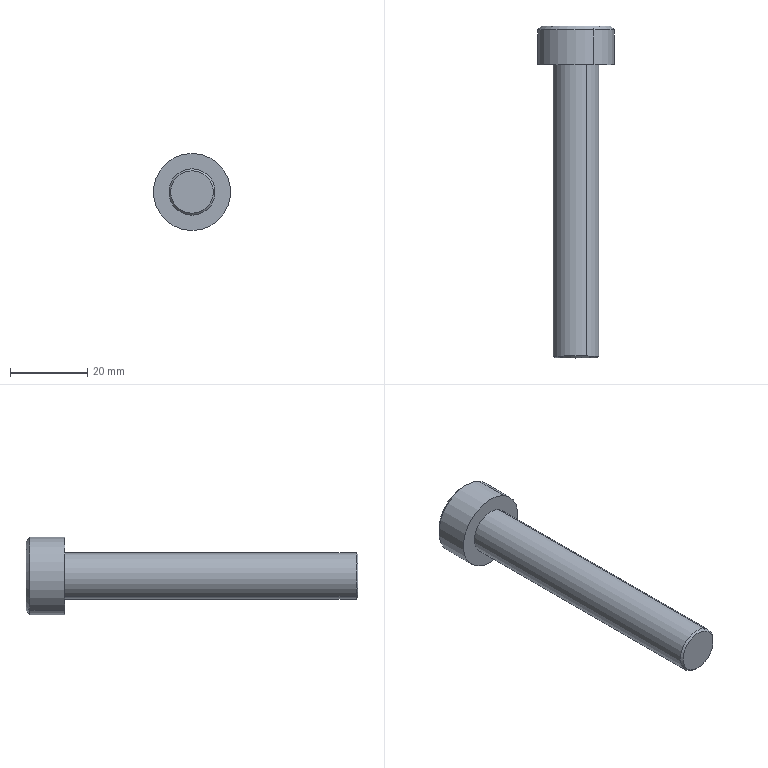Component | SolidWorks | DirectPressureVerticalSeal-1_PinShaft-1 | 1 solid | 11 faces | box 20 x 86 x 20 mm | volume 11702 mm3 | cylinder 4 | cone 4 | plane 3 | commonest cylinder face diameters 12 x2 20 x2
STEP:
#1=COLOUR_RGB('',0.7922,0.8196,0.9333);
#2=FILL_AREA_STYLE_COLOUR('',#1);
#3=FILL_AREA_STYLE('',(#2));
#4=SURFACE_STYLE_FILL_AREA(#3);
#5=SURFACE_SIDE_STYLE('',(#4));
#6=SURFACE_STYLE_USAGE(.BOTH.,#5);
#7=PRESENTATION_STYLE_ASSIGNMENT((#6));
#8=CARTESIAN_POINT('',(-4.959,8.243,11.567));
#9=VERTEX_POINT('',#8);
#10=CARTESIAN_POINT('',(-5.179,8.243,11.149));
#11=VERTEX_POINT('',#10);
#12=CARTESIAN_POINT('',(-5.069,8.243,11.358));
#13=DIRECTION('',(0.,1.,0.));
#14=DIRECTION('',(0.4655,0.,0.885));
#15=AXIS2_PLACEMENT_3D('',#12,#13,#14);
#16=CIRCLE('',#15,0.2362);
#17=EDGE_CURVE('',#9,#11,#16,.T.);
#18=ORIENTED_EDGE('',*,*,#17,.T.);
#19=CARTESIAN_POINT('',(-5.179,11.215,11.149));
#20=VERTEX_POINT('',#19);
#21=CARTESIAN_POINT('',(-5.179,11.609,11.149));
#22=DIRECTION('',(0.,1.,0.));
#23=VECTOR('',#22,39.37);
#24=LINE('',#21,#23);
#25=EDGE_CURVE('',#11,#20,#24,.T.);
#26=ORIENTED_EDGE('',*,*,#25,.T.);
#27=CARTESIAN_POINT('',(-4.959,11.215,11.567));
#28=VERTEX_POINT('',#27);
#29=CARTESIAN_POINT('',(-5.069,11.215,11.358));
#30=DIRECTION('',(-0.,-1.,-0.));
#31=DIRECTION('',(0.4655,0.,0.885));
#32=AXIS2_PLACEMENT_3D('',#29,#30,#31);
#33=CIRCLE('',#32,0.2362);
#34=EDGE_CURVE('',#20,#28,#33,.T.);
#35=ORIENTED_EDGE('',*,*,#34,.T.);
#36=CARTESIAN_POINT('',(-4.959,11.609,11.567));
#37=DIRECTION('',(0.,1.,0.));
#38=VECTOR('',#37,39.37);
#39=LINE('',#36,#38);
#40=EDGE_CURVE('',#9,#28,#39,.T.);
#41=ORIENTED_EDGE('',*,*,#40,.F.);
#42=EDGE_LOOP('',(#18,#26,#35,#41));
#43=FACE_OUTER_BOUND('',#42,.T.);
#44=CARTESIAN_POINT('',(-5.069,11.609,11.358));
#45=DIRECTION('',(0.,1.,0.));
#46=DIRECTION('',(0.4655,0.,0.885));
#47=AXIS2_PLACEMENT_3D('',#44,#45,#46);
#48=CYLINDRICAL_SURFACE('',#47,0.2362);
#49=ADVANCED_FACE('',(#43),#48,.T.);
#50=CARTESIAN_POINT('',(-4.968,8.223,11.55));
#51=VERTEX_POINT('',#50);
#52=CARTESIAN_POINT('',(-5.17,8.223,11.167));
#53=VERTEX_POINT('',#52);
#54=CARTESIAN_POINT('',(-5.069,8.223,11.358));
#55=DIRECTION('',(0.,1.,0.));
#56=DIRECTION('',(0.4655,0.,0.885));
#57=AXIS2_PLACEMENT_3D('',#54,#55,#56);
#58=CIRCLE('',#57,0.2165);
#59=EDGE_CURVE('',#51,#53,#58,.T.);
#60=ORIENTED_EDGE('',*,*,#59,.T.);
#61=CARTESIAN_POINT('',(-5.179,8.243,11.149));
#62=DIRECTION('',(-0.3292,0.7071,-0.6258));
#63=VECTOR('',#62,39.37);
#64=LINE('',#61,#63);
#65=EDGE_CURVE('',#53,#11,#64,.T.);
#66=ORIENTED_EDGE('',*,*,#65,.T.);
#67=ORIENTED_EDGE('',*,*,#17,.F.);
#68=CARTESIAN_POINT('',(-4.959,8.243,11.567));
#69=DIRECTION('',(0.3292,0.7071,0.6258));
#70=VECTOR('',#69,39.37);
#71=LINE('',#68,#70);
#72=EDGE_CURVE('',#51,#9,#71,.T.);
#73=ORIENTED_EDGE('',*,*,#72,.F.);
#74=EDGE_LOOP('',(#60,#66,#67,#73));
#75=FACE_OUTER_BOUND('',#74,.T.);
#76=CARTESIAN_POINT('',(-5.069,8.243,11.358));
#77=DIRECTION('',(0.,1.,0.));
#78=DIRECTION('',(0.4655,0.,0.885));
#79=AXIS2_PLACEMENT_3D('',#76,#77,#78);
#80=CONICAL_SURFACE('',#79,0.2362,0.7854);
#81=ADVANCED_FACE('',(#75),#80,.T.);
#82=CARTESIAN_POINT('',(-4.885,11.215,11.707));
#83=VERTEX_POINT('',#82);
#84=CARTESIAN_POINT('',(-5.252,11.215,11.01));
#85=VERTEX_POINT('',#84);
#86=CARTESIAN_POINT('',(-5.069,11.215,11.358));
#87=DIRECTION('',(0.,1.,0.));
#88=DIRECTION('',(0.4655,0.,0.885));
#89=AXIS2_PLACEMENT_3D('',#86,#87,#88);
#90=CIRCLE('',#89,0.3937);
#91=EDGE_CURVE('',#83,#85,#90,.T.);
#92=ORIENTED_EDGE('',*,*,#91,.T.);
#93=CARTESIAN_POINT('',(-5.252,11.57,11.01));
#94=VERTEX_POINT('',#93);
#95=CARTESIAN_POINT('',(-5.252,11.609,11.01));
#96=DIRECTION('',(0.,1.,0.));
#97=VECTOR('',#96,39.37);
#98=LINE('',#95,#97);
#99=EDGE_CURVE('',#85,#94,#98,.T.);
#100=ORIENTED_EDGE('',*,*,#99,.T.);
#101=CARTESIAN_POINT('',(-4.885,11.57,11.707));
#102=VERTEX_POINT('',#101);
#103=CARTESIAN_POINT('',(-5.069,11.57,11.358));
#104=DIRECTION('',(-0.,-1.,-0.));
#105=DIRECTION('',(0.4655,0.,0.885));
#106=AXIS2_PLACEMENT_3D('',#103,#104,#105);
#107=CIRCLE('',#106,0.3937);
#108=EDGE_CURVE('',#94,#102,#107,.T.);
#109=ORIENTED_EDGE('',*,*,#108,.T.);
#110=CARTESIAN_POINT('',(-4.885,11.609,11.707));
#111=DIRECTION('',(0.,1.,0.));
#112=VECTOR('',#111,39.37);
#113=LINE('',#110,#112);
#114=EDGE_CURVE('',#83,#102,#113,.T.);
#115=ORIENTED_EDGE('',*,*,#114,.F.);
#116=EDGE_LOOP('',(#92,#100,#109,#115));
#117=FACE_OUTER_BOUND('',#116,.T.);
#118=CARTESIAN_POINT('',(-5.069,11.609,11.358));
#119=DIRECTION('',(0.,1.,0.));
#120=DIRECTION('',(0.4655,0.,0.885));
#121=AXIS2_PLACEMENT_3D('',#118,#119,#120);
#122=CYLINDRICAL_SURFACE('',#121,0.3937);
#123=ADVANCED_FACE('',(#117),#122,.T.);
#124=CARTESIAN_POINT('',(-5.234,11.609,11.045));
#125=VERTEX_POINT('',#124);
#126=CARTESIAN_POINT('',(-4.904,11.609,11.672));
#127=VERTEX_POINT('',#126);
#128=CARTESIAN_POINT('',(-5.069,11.609,11.358));
#129=DIRECTION('',(-0.,-1.,-0.));
#130=DIRECTION('',(-0.4655,0.,-0.885));
#131=AXIS2_PLACEMENT_3D('',#128,#129,#130);
#132=CIRCLE('',#131,0.3543);
#133=EDGE_CURVE('',#125,#127,#132,.T.);
#134=ORIENTED_EDGE('',*,*,#133,.T.);
#135=CARTESIAN_POINT('',(-4.885,11.57,11.707));
#136=DIRECTION('',(0.3292,-0.7071,0.6258));
#137=VECTOR('',#136,39.37);
#138=LINE('',#135,#137);
#139=EDGE_CURVE('',#127,#102,#138,.T.);
#140=ORIENTED_EDGE('',*,*,#139,.T.);
#141=ORIENTED_EDGE('',*,*,#108,.F.);
#142=CARTESIAN_POINT('',(-5.252,11.57,11.01));
#143=DIRECTION('',(-0.3292,-0.7071,-0.6258));
#144=VECTOR('',#143,39.37);
#145=LINE('',#142,#144);
#146=EDGE_CURVE('',#125,#94,#145,.T.);
#147=ORIENTED_EDGE('',*,*,#146,.F.);
#148=EDGE_LOOP('',(#134,#140,#141,#147));
#149=FACE_OUTER_BOUND('',#148,.T.);
#150=CARTESIAN_POINT('',(-5.069,11.57,11.358));
#151=DIRECTION('',(-0.,-1.,-0.));
#152=DIRECTION('',(-0.4655,0.,-0.885));
#153=AXIS2_PLACEMENT_3D('',#150,#151,#152);
#154=CONICAL_SURFACE('',#153,0.3937,0.7854);
#155=ADVANCED_FACE('',(#149),#154,.T.);
#156=ORIENTED_EDGE('',*,*,#25,.F.);
#157=CARTESIAN_POINT('',(-5.069,8.243,11.358));
#158=DIRECTION('',(0.,1.,0.));
#159=DIRECTION('',(0.4655,0.,0.885));
#160=AXIS2_PLACEMENT_3D('',#157,#158,#159);
#161=CIRCLE('',#160,0.2362);
#162=EDGE_CURVE('',#11,#9,#161,.T.);
#163=ORIENTED_EDGE('',*,*,#162,.T.);
#164=ORIENTED_EDGE('',*,*,#40,.T.);
#165=CARTESIAN_POINT('',(-5.069,11.215,11.358));
#166=DIRECTION('',(-0.,-1.,-0.));
#167=DIRECTION('',(0.4655,0.,0.885));
#168=AXIS2_PLACEMENT_3D('',#165,#166,#167);
#169=CIRCLE('',#168,0.2362);
#170=EDGE_CURVE('',#28,#20,#169,.T.);
#171=ORIENTED_EDGE('',*,*,#170,.T.);
#172=EDGE_LOOP('',(#156,#163,#164,#171));
#173=FACE_OUTER_BOUND('',#172,.T.);
#174=CARTESIAN_POINT('',(-5.069,11.609,11.358));
#175=DIRECTION('',(0.,1.,0.));
#176=DIRECTION('',(0.4655,0.,0.885));
#177=AXIS2_PLACEMENT_3D('',#174,#175,#176);
#178=CYLINDRICAL_SURFACE('',#177,0.2362);
#179=ADVANCED_FACE('',(#173),#178,.T.);
#180=ORIENTED_EDGE('',*,*,#91,.F.);
#181=CARTESIAN_POINT('',(-5.069,11.215,11.358));
#182=DIRECTION('',(0.,1.,0.));
#183=DIRECTION('',(0.4655,0.,0.885));
#184=AXIS2_PLACEMENT_3D('',#181,#182,#183);
#185=CIRCLE('',#184,0.3937);
#186=EDGE_CURVE('',#85,#83,#185,.T.);
#187=ORIENTED_EDGE('',*,*,#186,.F.);
#188=EDGE_LOOP('',(#180,#187));
#189=FACE_OUTER_BOUND('',#188,.T.);
#190=ORIENTED_EDGE('',*,*,#170,.F.);
#191=ORIENTED_EDGE('',*,*,#34,.F.);
#192=EDGE_LOOP('',(#190,#191));
#193=FACE_BOUND('',#192,.T.);
#194=CARTESIAN_POINT('',(-4.86,11.215,11.248));
#195=DIRECTION('',(0.,1.,0.));
#196=DIRECTION('',(0.4655,-0.,0.885));
#197=AXIS2_PLACEMENT_3D('',#194,#195,#196);
#198=PLANE('',#197);
#199=ADVANCED_FACE('',(#189,#193),#198,.F.);
#200=ORIENTED_EDGE('',*,*,#65,.F.);
#201=CARTESIAN_POINT('',(-5.069,8.223,11.358));
#202=DIRECTION('',(0.,1.,0.));
#203=DIRECTION('',(0.4655,0.,0.885));
#204=AXIS2_PLACEMENT_3D('',#201,#202,#203);
#205=CIRCLE('',#204,0.2165);
#206=EDGE_CURVE('',#53,#51,#205,.T.);
#207=ORIENTED_EDGE('',*,*,#206,.T.);
#208=ORIENTED_EDGE('',*,*,#72,.T.);
#209=ORIENTED_EDGE('',*,*,#162,.F.);
#210=EDGE_LOOP('',(#200,#207,#208,#209));
#211=FACE_OUTER_BOUND('',#210,.T.);
#212=CARTESIAN_POINT('',(-5.069,8.243,11.358));
#213=DIRECTION('',(0.,1.,0.));
#214=DIRECTION('',(0.4655,0.,0.885));
#215=AXIS2_PLACEMENT_3D('',#212,#213,#214);
#216=CONICAL_SURFACE('',#215,0.2362,0.7854);
#217=ADVANCED_FACE('',(#211),#216,.T.);
#218=ORIENTED_EDGE('',*,*,#99,.F.);
#219=ORIENTED_EDGE('',*,*,#186,.T.);
#220=ORIENTED_EDGE('',*,*,#114,.T.);
#221=CARTESIAN_POINT('',(-5.069,11.57,11.358));
#222=DIRECTION('',(-0.,-1.,-0.));
#223=DIRECTION('',(0.4655,0.,0.885));
#224=AXIS2_PLACEMENT_3D('',#221,#222,#223);
#225=CIRCLE('',#224,0.3937);
#226=EDGE_CURVE('',#102,#94,#225,.T.);
#227=ORIENTED_EDGE('',*,*,#226,.T.);
#228=EDGE_LOOP('',(#218,#219,#220,#227));
#229=FACE_OUTER_BOUND('',#228,.T.);
#230=CARTESIAN_POINT('',(-5.069,11.609,11.358));
#231=DIRECTION('',(0.,1.,0.));
#232=DIRECTION('',(0.4655,0.,0.885));
#233=AXIS2_PLACEMENT_3D('',#230,#231,#232);
#234=CYLINDRICAL_SURFACE('',#233,0.3937);
#235=ADVANCED_FACE('',(#229),#234,.T.);
#236=ORIENTED_EDGE('',*,*,#59,.F.);
#237=ORIENTED_EDGE('',*,*,#206,.F.);
#238=EDGE_LOOP('',(#236,#237));
#239=FACE_OUTER_BOUND('',#238,.T.);
#240=CARTESIAN_POINT('',(-5.069,8.223,11.358));
#241=DIRECTION('',(0.,1.,0.));
#242=DIRECTION('',(0.4655,-0.,0.885));
#243=AXIS2_PLACEMENT_3D('',#240,#241,#242);
#244=PLANE('',#243);
#245=ADVANCED_FACE('',(#239),#244,.F.);
#246=ORIENTED_EDGE('',*,*,#139,.F.);
#247=CARTESIAN_POINT('',(-5.069,11.609,11.358));
#248=DIRECTION('',(-0.,-1.,-0.));
#249=DIRECTION('',(-0.4655,0.,-0.885));
#250=AXIS2_PLACEMENT_3D('',#247,#248,#249);
#251=CIRCLE('',#250,0.3543);
#252=EDGE_CURVE('',#127,#125,#251,.T.);
#253=ORIENTED_EDGE('',*,*,#252,.T.);
#254=ORIENTED_EDGE('',*,*,#146,.T.);
#255=ORIENTED_EDGE('',*,*,#226,.F.);
#256=EDGE_LOOP('',(#246,#253,#254,#255));
#257=FACE_OUTER_BOUND('',#256,.T.);
#258=CARTESIAN_POINT('',(-5.069,11.57,11.358));
#259=DIRECTION('',(-0.,-1.,-0.));
#260=DIRECTION('',(-0.4655,0.,-0.885));
#261=AXIS2_PLACEMENT_3D('',#258,#259,#260);
#262=CONICAL_SURFACE('',#261,0.3937,0.7854);
#263=ADVANCED_FACE('',(#257),#262,.T.);
#264=ORIENTED_EDGE('',*,*,#133,.F.);
#265=ORIENTED_EDGE('',*,*,#252,.F.);
#266=EDGE_LOOP('',(#264,#265));
#267=FACE_OUTER_BOUND('',#266,.T.);
#268=CARTESIAN_POINT('',(-4.755,11.609,11.193));
#269=DIRECTION('',(-0.,-1.,-0.));
#270=DIRECTION('',(-0.4655,0.,-0.885));
#271=AXIS2_PLACEMENT_3D('',#268,#269,#270);
#272=PLANE('',#271);
#273=ADVANCED_FACE('',(#267),#272,.F.);
#274=CLOSED_SHELL('',(#49,#81,#123,#155,#179,#199,#217,#235,#245,#263,#273));
#275=MANIFOLD_SOLID_BREP('',#274);
#276=STYLED_ITEM('',(#7),#275);
#277=(LENGTH_UNIT()NAMED_UNIT(*)SI_UNIT($,.METRE.));
#278=LENGTH_MEASURE_WITH_UNIT(LENGTH_MEASURE(0.0254),#277);
#279=DIMENSIONAL_EXPONENTS(1.,0.,0.,0.,0.,0.,0.);
#280=(CONVERSION_BASED_UNIT('',#278)LENGTH_UNIT()NAMED_UNIT(#279));
#281=UNCERTAINTY_MEASURE_WITH_UNIT(LENGTH_MEASURE(0.00001),#280,'','');
#282=(NAMED_UNIT(*)PLANE_ANGLE_UNIT()SI_UNIT($,.RADIAN.));
#283=(NAMED_UNIT(*)SI_UNIT($,.STERADIAN.)SOLID_ANGLE_UNIT());
#284=(GEOMETRIC_REPRESENTATION_CONTEXT(3)GLOBAL_UNCERTAINTY_ASSIGNED_CONTEXT((#281))GLOBAL_UNIT_ASSIGNED_CONTEXT((#280,#282,#283))REPRESENTATION_CONTEXT('',''));
#285=MECHANICAL_DESIGN_GEOMETRIC_PRESENTATION_REPRESENTATION('',(#276),#284);
#286=CARTESIAN_POINT('',(0.,0.,0.));
#287=DIRECTION('',(0.,0.,1.));
#288=DIRECTION('',(1.,0.,0.));
#289=AXIS2_PLACEMENT_3D('',#286,#287,#288);
#290=(LENGTH_UNIT()NAMED_UNIT(*)SI_UNIT($,.METRE.));
#291=LENGTH_MEASURE_WITH_UNIT(LENGTH_MEASURE(0.0254),#290);
#292=DIMENSIONAL_EXPONENTS(1.,0.,0.,0.,0.,0.,0.);
#293=(CONVERSION_BASED_UNIT('',#291)LENGTH_UNIT()NAMED_UNIT(#292));
#294=UNCERTAINTY_MEASURE_WITH_UNIT(LENGTH_MEASURE(0.00001),#293,'','');
#295=(NAMED_UNIT(*)PLANE_ANGLE_UNIT()SI_UNIT($,.RADIAN.));
#296=(NAMED_UNIT(*)SI_UNIT($,.STERADIAN.)SOLID_ANGLE_UNIT());
#297=(GEOMETRIC_REPRESENTATION_CONTEXT(3)GLOBAL_UNCERTAINTY_ASSIGNED_CONTEXT((#294))GLOBAL_UNIT_ASSIGNED_CONTEXT((#293,#295,#296))REPRESENTATION_CONTEXT('',''));
#298=ADVANCED_BREP_SHAPE_REPRESENTATION('',(#275,#289),#297);
#299=PRESENTATION_LAYER_ASSIGNMENT('','',(#276));